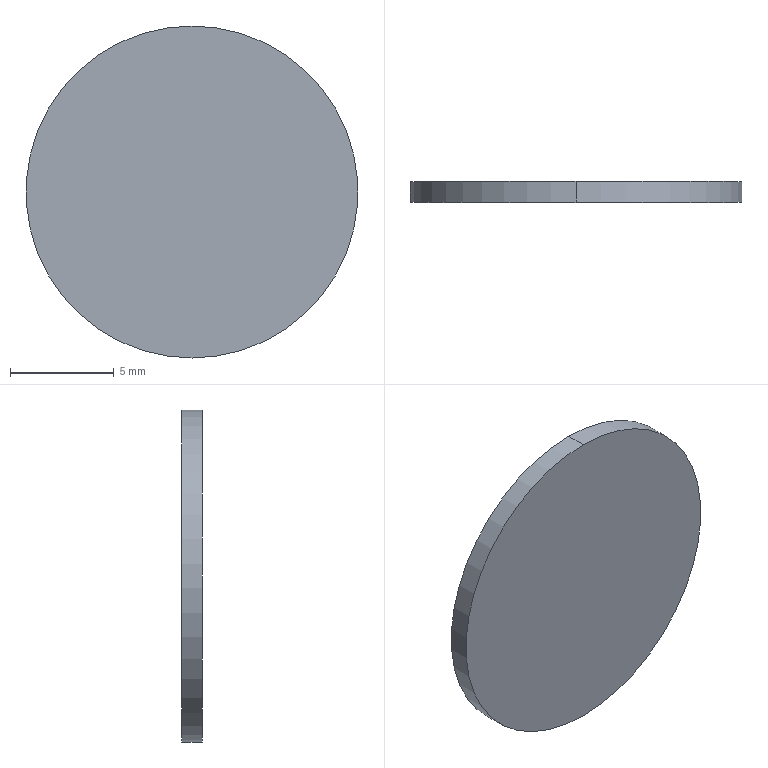Component | SolidWorks | CoolingPlateCover-1 | 1 solid | 4 faces | box 16 x 1 x 16 mm | volume 201 mm3 | cylinder 2 | plane 2 | commonest cylinder face diameters 16 x2
build123d program:
from build123d import *

# Parameters (mm, degrees)
SKETCH1_R           = 8
BOSS_EXTRUDE1_DEPTH = 1


with BuildPart() as part:
    # Sketch1 → Boss-Extrude1 (new body)
    with BuildSketch(Plane(origin=(0, 0, 0), x_dir=(1, 0, 0), z_dir=(0, 1, 0))):
        with Locations(Location((0, 0, 0), (0, 0, 270))):
            Circle(SKETCH1_R)
    extrude(amount=BOSS_EXTRUDE1_DEPTH)


solid = part.part

# Placed as in the assembly
solid = solid.moved(Location((-5.981, 20.506, 160), (0, 0, 0)))
STEP:
#1=COLOUR_RGB('',0.7922,0.8196,0.9333);
#2=FILL_AREA_STYLE_COLOUR('',#1);
#3=FILL_AREA_STYLE('',(#2));
#4=SURFACE_STYLE_FILL_AREA(#3);
#5=SURFACE_SIDE_STYLE('',(#4));
#6=SURFACE_STYLE_USAGE(.BOTH.,#5);
#7=PRESENTATION_STYLE_ASSIGNMENT((#6));
#8=CARTESIAN_POINT('',(-0.2355,0.8467,6.614));
#9=VERTEX_POINT('',#8);
#10=CARTESIAN_POINT('',(-0.2355,0.8467,5.984));
#11=VERTEX_POINT('',#10);
#12=CARTESIAN_POINT('',(-0.2355,0.8467,6.299));
#13=DIRECTION('',(0.,1.,0.));
#14=DIRECTION('',(0.,0.,1.));
#15=AXIS2_PLACEMENT_3D('',#12,#13,#14);
#16=CIRCLE('',#15,0.315);
#17=EDGE_CURVE('',#9,#11,#16,.T.);
#18=ORIENTED_EDGE('',*,*,#17,.F.);
#19=CARTESIAN_POINT('',(-0.2355,0.8073,6.614));
#20=VERTEX_POINT('',#19);
#21=CARTESIAN_POINT('',(-0.2355,0.8467,6.614));
#22=DIRECTION('',(0.,-1.,0.));
#23=VECTOR('',#22,39.37);
#24=LINE('',#21,#23);
#25=EDGE_CURVE('',#9,#20,#24,.T.);
#26=ORIENTED_EDGE('',*,*,#25,.T.);
#27=CARTESIAN_POINT('',(-0.2355,0.8073,5.984));
#28=VERTEX_POINT('',#27);
#29=CARTESIAN_POINT('',(-0.2355,0.8073,6.299));
#30=DIRECTION('',(0.,1.,0.));
#31=DIRECTION('',(0.,0.,1.));
#32=AXIS2_PLACEMENT_3D('',#29,#30,#31);
#33=CIRCLE('',#32,0.315);
#34=EDGE_CURVE('',#20,#28,#33,.T.);
#35=ORIENTED_EDGE('',*,*,#34,.T.);
#36=CARTESIAN_POINT('',(-0.2355,0.8467,5.984));
#37=DIRECTION('',(0.,-1.,0.));
#38=VECTOR('',#37,39.37);
#39=LINE('',#36,#38);
#40=EDGE_CURVE('',#11,#28,#39,.T.);
#41=ORIENTED_EDGE('',*,*,#40,.F.);
#42=EDGE_LOOP('',(#18,#26,#35,#41));
#43=FACE_OUTER_BOUND('',#42,.T.);
#44=CARTESIAN_POINT('',(-0.2355,0.8467,6.299));
#45=DIRECTION('',(0.,-1.,0.));
#46=DIRECTION('',(0.,0.,-1.));
#47=AXIS2_PLACEMENT_3D('',#44,#45,#46);
#48=CYLINDRICAL_SURFACE('',#47,0.315);
#49=ADVANCED_FACE('',(#43),#48,.T.);
#50=ORIENTED_EDGE('',*,*,#25,.F.);
#51=CARTESIAN_POINT('',(-0.2355,0.8467,6.299));
#52=DIRECTION('',(0.,1.,0.));
#53=DIRECTION('',(0.,0.,1.));
#54=AXIS2_PLACEMENT_3D('',#51,#52,#53);
#55=CIRCLE('',#54,0.315);
#56=EDGE_CURVE('',#11,#9,#55,.T.);
#57=ORIENTED_EDGE('',*,*,#56,.F.);
#58=ORIENTED_EDGE('',*,*,#40,.T.);
#59=CARTESIAN_POINT('',(-0.2355,0.8073,6.299));
#60=DIRECTION('',(0.,1.,0.));
#61=DIRECTION('',(0.,0.,1.));
#62=AXIS2_PLACEMENT_3D('',#59,#60,#61);
#63=CIRCLE('',#62,0.315);
#64=EDGE_CURVE('',#28,#20,#63,.T.);
#65=ORIENTED_EDGE('',*,*,#64,.T.);
#66=EDGE_LOOP('',(#50,#57,#58,#65));
#67=FACE_OUTER_BOUND('',#66,.T.);
#68=CARTESIAN_POINT('',(-0.2355,0.8467,6.299));
#69=DIRECTION('',(0.,-1.,0.));
#70=DIRECTION('',(0.,0.,-1.));
#71=AXIS2_PLACEMENT_3D('',#68,#69,#70);
#72=CYLINDRICAL_SURFACE('',#71,0.315);
#73=ADVANCED_FACE('',(#67),#72,.T.);
#74=ORIENTED_EDGE('',*,*,#56,.T.);
#75=ORIENTED_EDGE('',*,*,#17,.T.);
#76=EDGE_LOOP('',(#74,#75));
#77=FACE_OUTER_BOUND('',#76,.T.);
#78=CARTESIAN_POINT('',(-0.2355,0.8467,6.299));
#79=DIRECTION('',(0.,1.,0.));
#80=DIRECTION('',(0.,0.,1.));
#81=AXIS2_PLACEMENT_3D('',#78,#79,#80);
#82=PLANE('',#81);
#83=ADVANCED_FACE('',(#77),#82,.T.);
#84=ORIENTED_EDGE('',*,*,#64,.F.);
#85=ORIENTED_EDGE('',*,*,#34,.F.);
#86=EDGE_LOOP('',(#84,#85));
#87=FACE_OUTER_BOUND('',#86,.T.);
#88=CARTESIAN_POINT('',(-0.2355,0.8073,6.299));
#89=DIRECTION('',(0.,1.,0.));
#90=DIRECTION('',(0.,0.,1.));
#91=AXIS2_PLACEMENT_3D('',#88,#89,#90);
#92=PLANE('',#91);
#93=ADVANCED_FACE('',(#87),#92,.F.);
#94=CLOSED_SHELL('',(#49,#73,#83,#93));
#95=MANIFOLD_SOLID_BREP('',#94);
#96=STYLED_ITEM('',(#7),#95);
#97=PRESENTATION_LAYER_ASSIGNMENT('','',(#96));
#98=CARTESIAN_POINT('',(0.,0.,0.));
#99=DIRECTION('',(0.,0.,1.));
#100=DIRECTION('',(1.,0.,0.));
#101=AXIS2_PLACEMENT_3D('',#98,#99,#100);
#102=(LENGTH_UNIT()NAMED_UNIT(*)SI_UNIT($,.METRE.));
#103=LENGTH_MEASURE_WITH_UNIT(LENGTH_MEASURE(0.0254),#102);
#104=DIMENSIONAL_EXPONENTS(1.,0.,0.,0.,0.,0.,0.);
#105=(CONVERSION_BASED_UNIT('',#103)LENGTH_UNIT()NAMED_UNIT(#104));
#106=UNCERTAINTY_MEASURE_WITH_UNIT(LENGTH_MEASURE(0.00001),#105,'','');
#107=(NAMED_UNIT(*)PLANE_ANGLE_UNIT()SI_UNIT($,.RADIAN.));
#108=(NAMED_UNIT(*)SI_UNIT($,.STERADIAN.)SOLID_ANGLE_UNIT());
#109=(GEOMETRIC_REPRESENTATION_CONTEXT(3)GLOBAL_UNCERTAINTY_ASSIGNED_CONTEXT((#106))GLOBAL_UNIT_ASSIGNED_CONTEXT((#105,#107,#108))REPRESENTATION_CONTEXT('',''));
#110=ADVANCED_BREP_SHAPE_REPRESENTATION('',(#95,#101),#109);
#111=(LENGTH_UNIT()NAMED_UNIT(*)SI_UNIT($,.METRE.));
#112=LENGTH_MEASURE_WITH_UNIT(LENGTH_MEASURE(0.0254),#111);
#113=DIMENSIONAL_EXPONENTS(1.,0.,0.,0.,0.,0.,0.);
#114=(CONVERSION_BASED_UNIT('',#112)LENGTH_UNIT()NAMED_UNIT(#113));
#115=UNCERTAINTY_MEASURE_WITH_UNIT(LENGTH_MEASURE(0.00001),#114,'','');
#116=(NAMED_UNIT(*)PLANE_ANGLE_UNIT()SI_UNIT($,.RADIAN.));
#117=(NAMED_UNIT(*)SI_UNIT($,.STERADIAN.)SOLID_ANGLE_UNIT());
#118=(GEOMETRIC_REPRESENTATION_CONTEXT(3)GLOBAL_UNCERTAINTY_ASSIGNED_CONTEXT((#115))GLOBAL_UNIT_ASSIGNED_CONTEXT((#114,#116,#117))REPRESENTATION_CONTEXT('',''));
#119=MECHANICAL_DESIGN_GEOMETRIC_PRESENTATION_REPRESENTATION('',(#96),#118);